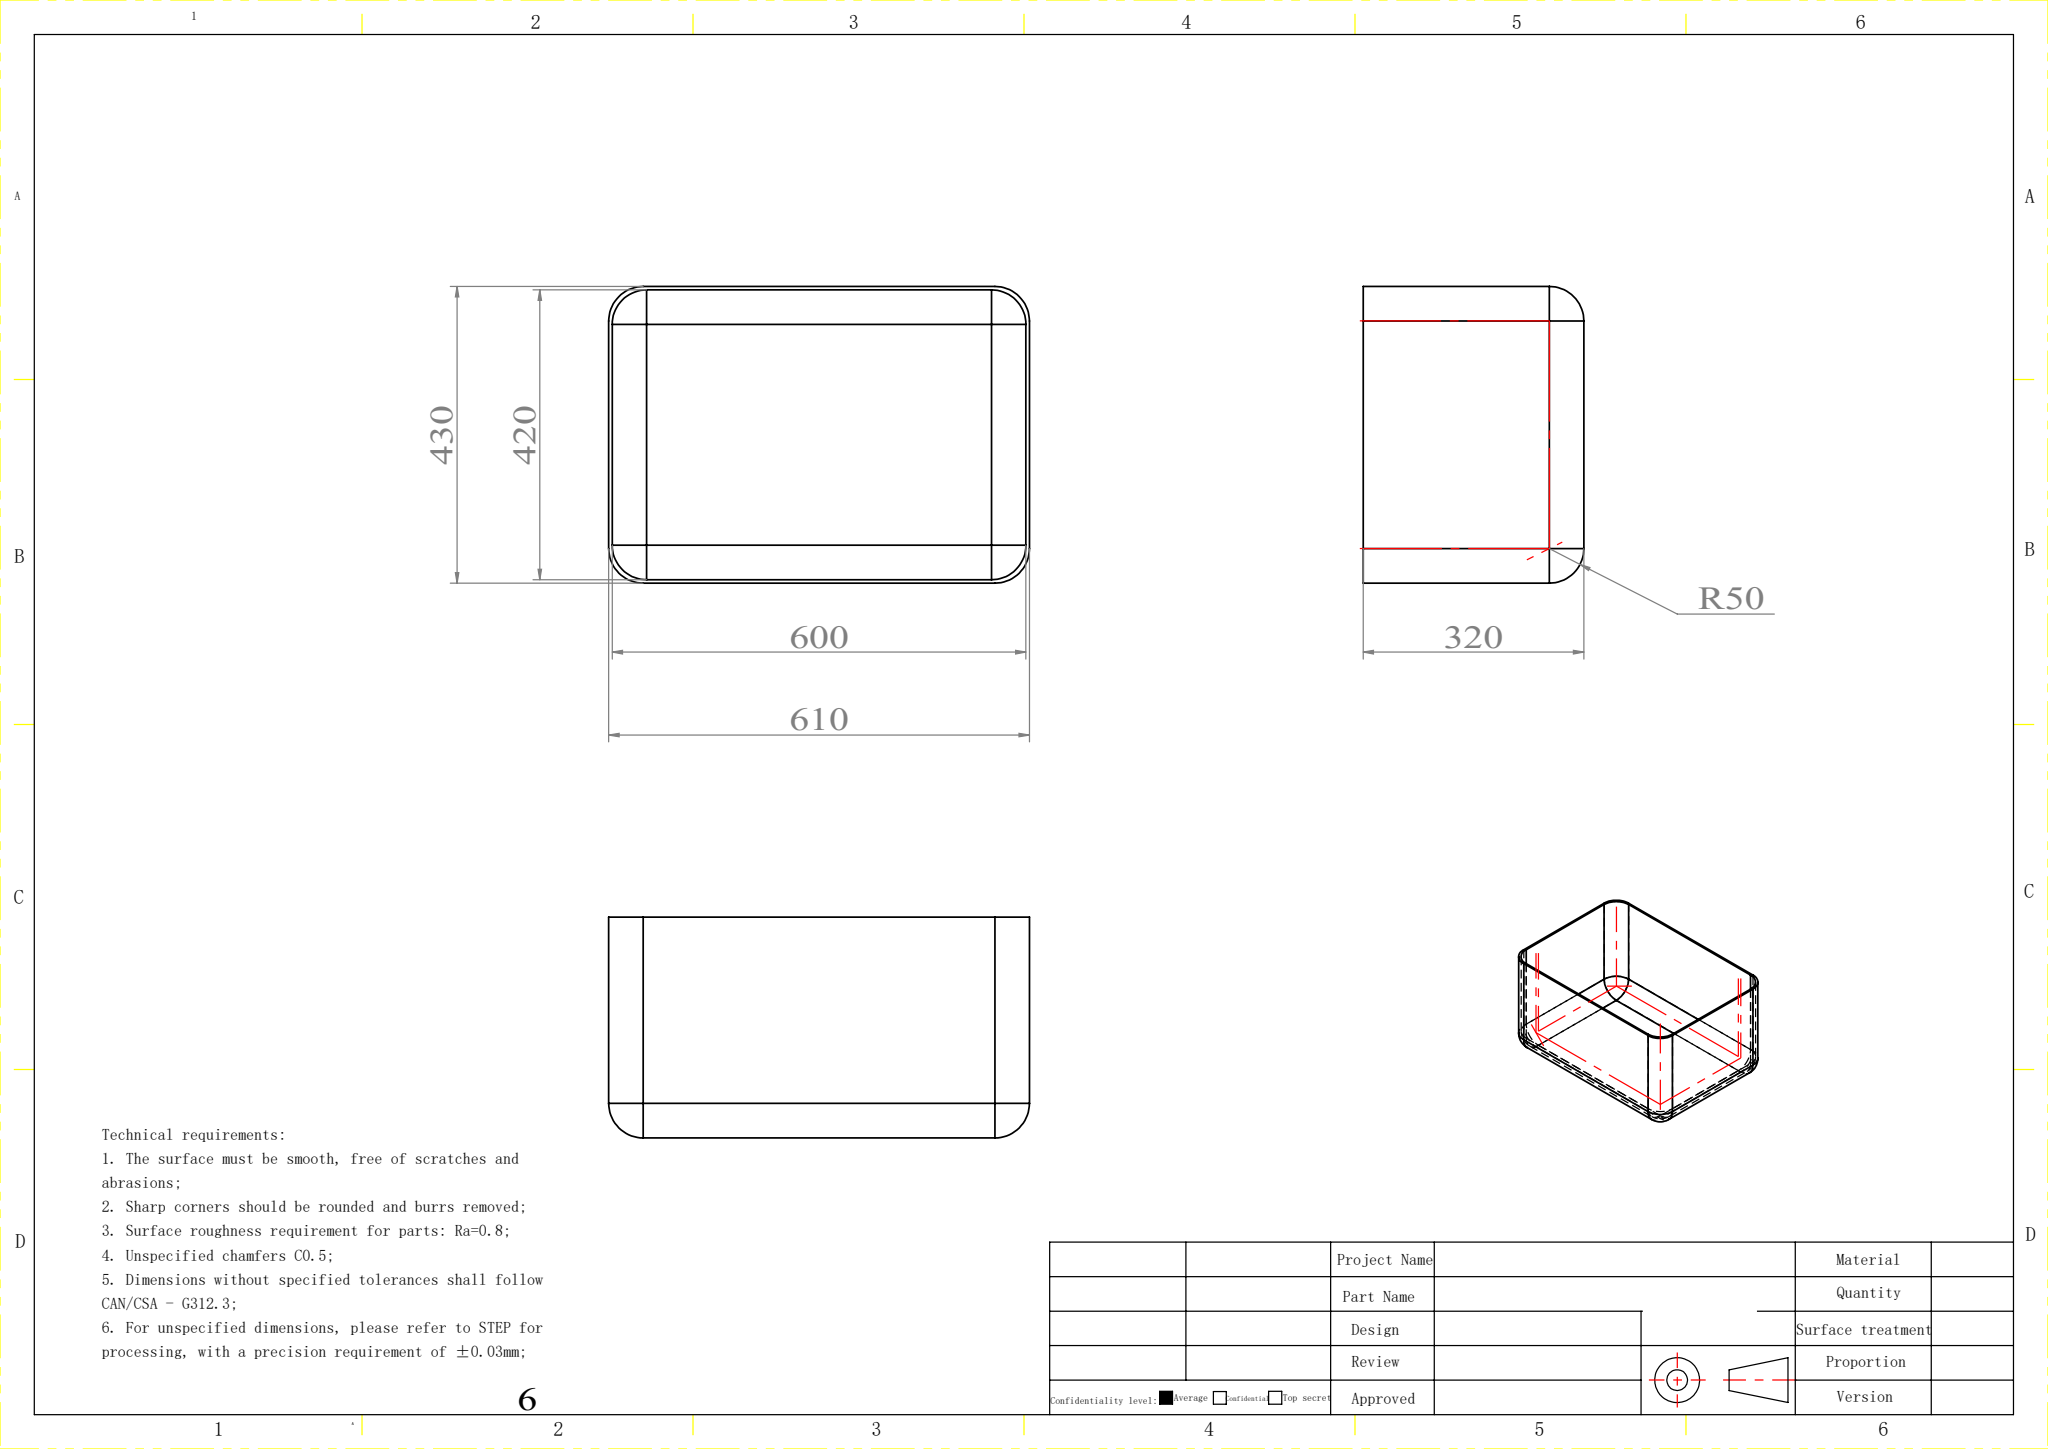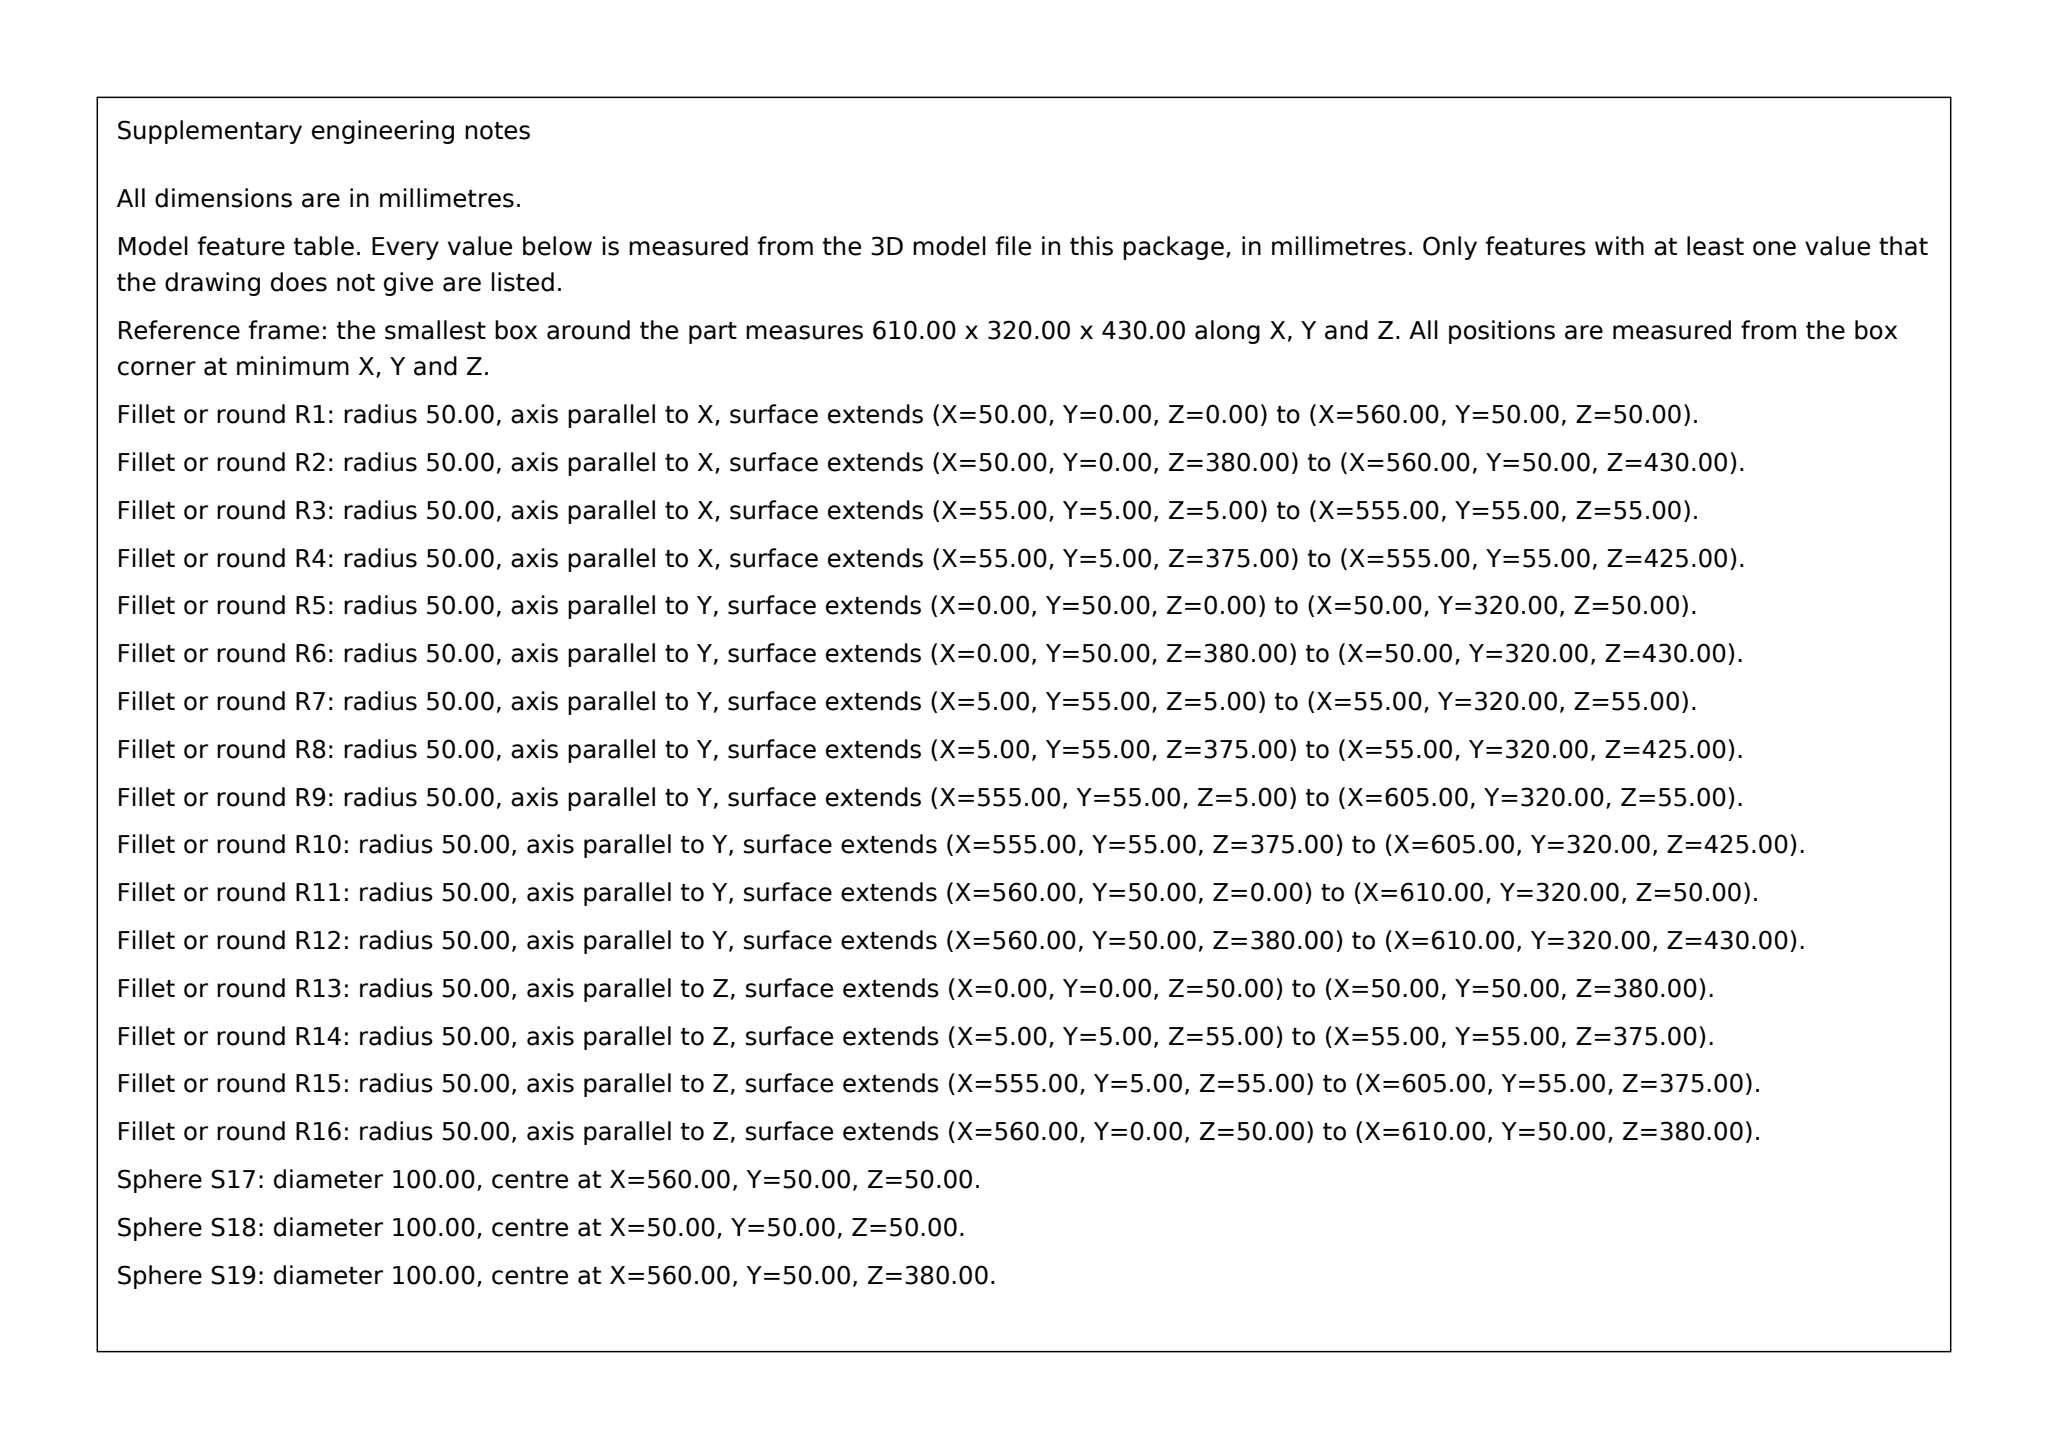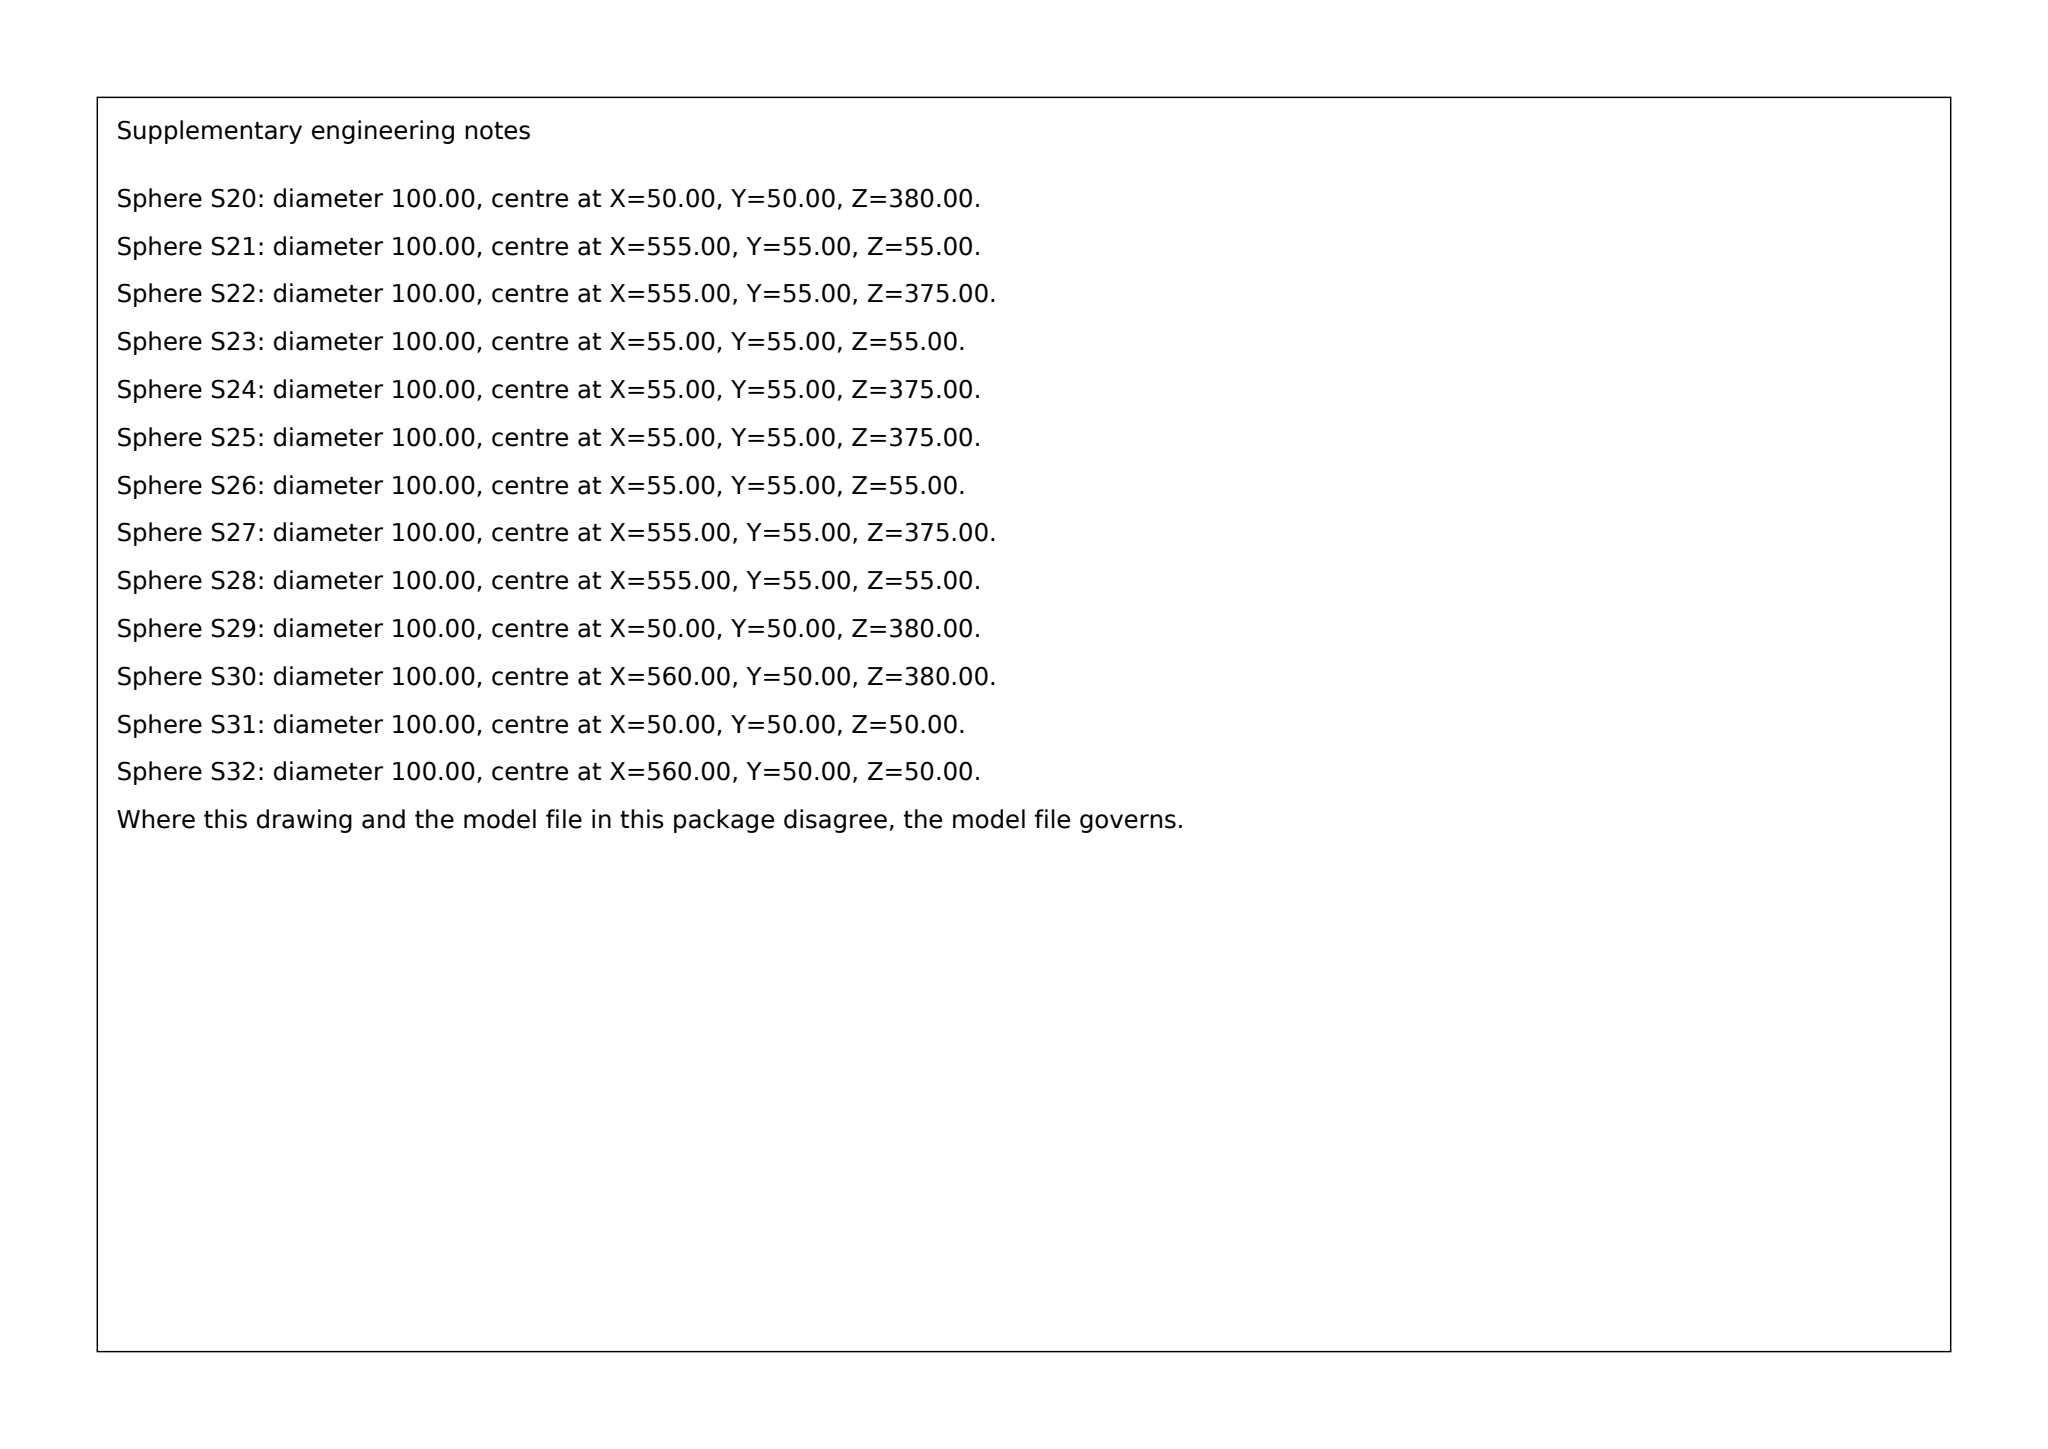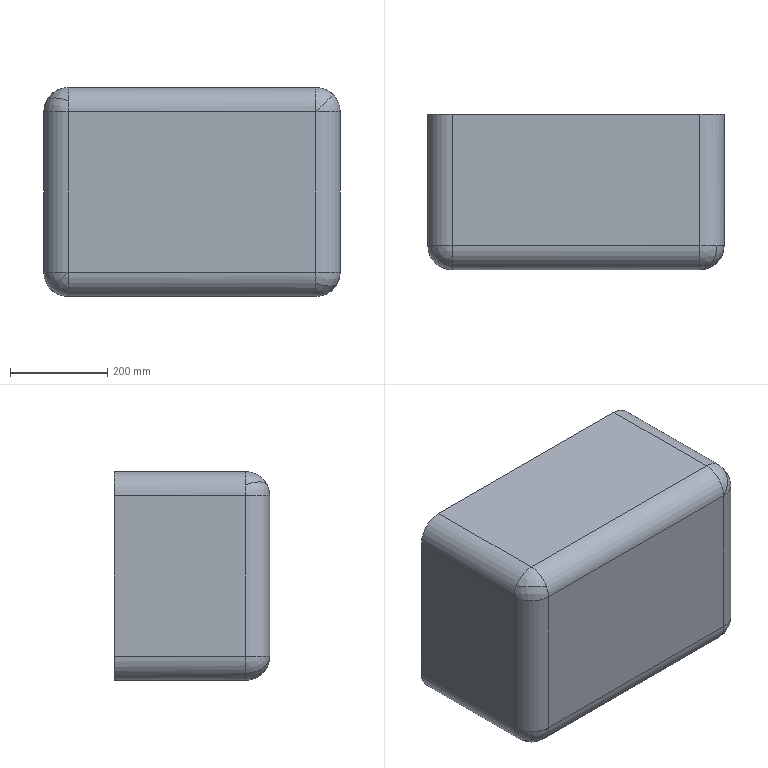Part | SolidWorks | mm | 1 solid | 43 faces | box 610 x 320 x 430 mm | volume 4523810 mm3 | sphere 16 | cylinder 16 | plane 11 | commonest cylinder face diameters 100 x16